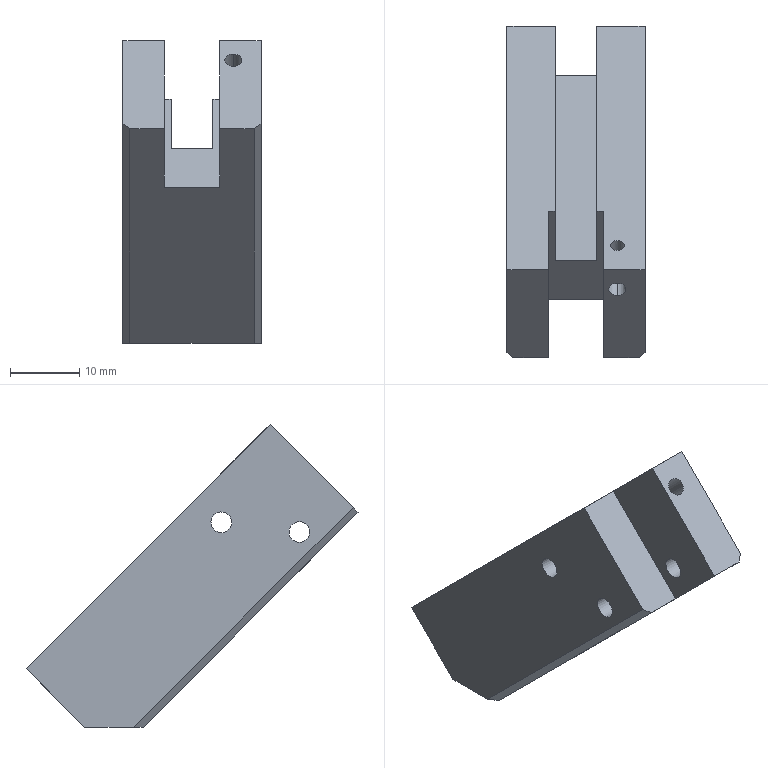Component | SolidWorks | ZL-10-07Slider-1 | 1 solid | 34 faces | box 20 x 48.08 x 43.84 mm | volume 13354 mm3 | plane 18 | cylinder 14 | cone 2 | commonest cylinder face diameters 3 x8 2 x4 2.5 x2
build123d program:
from build123d import *

# Parameters (mm, degrees)
EXTRUDE1_DEPTH        = 50
M3_TAPPED_HOLE1_D     = 2.5
M3_TAPPED_HOLE1_DEPTH = 7.5
M3_TAPPED_HOLE1_TIP   = 0.7511
SKETCH6_R             = 1
CUT_EXTRUDE1_DEPTH    = 6
CHAMFER1_SIZE         = 6
SKETCH7_R             = 1.5
CUT_EXTRUDE2_DEPTH    = 57.78
SKETCH8_W             = 8
SKETCH8_H             = 12
CUT_EXTRUDE3_DEPTH    = 55.074
SKETCH9_R             = 1.5
CUT_EXTRUDE4_DEPTH    = 57.78
CHAMFER2_SIZE         = 1


with BuildPart() as part:
    # Sketch1 → Extrude1 (new body)
    with BuildSketch(Plane(origin=(0, 0, 0), x_dir=(1, 0, 0), z_dir=(0, 1, 0))):
        Polygon((10, 0), (-10, 0), (-10, 18), (-3, 18), (-3, 8), (3, 8), (3, 18), (10, 18), align=None)
    extrude(amount=EXTRUDE1_DEPTH)

    # M3 Tapped Hole1
    with Locations(Plane.XZ):
        with Locations((-6, -14)):
            Hole(M3_TAPPED_HOLE1_D / 2, depth=M3_TAPPED_HOLE1_DEPTH)
            with Locations((0, 0, -(M3_TAPPED_HOLE1_DEPTH + M3_TAPPED_HOLE1_TIP / 2))):  # 118° drill point
                Cone(0, M3_TAPPED_HOLE1_D / 2, M3_TAPPED_HOLE1_TIP, mode=Mode.SUBTRACT)

    # Sketch6 → Cut-Extrude1 (cut)
    with BuildSketch(Plane(origin=(0, 0, -18), x_dir=(-1, 0, 0), z_dir=(0, 0, -1))):
        with Locations((6, 5)):
            Circle(SKETCH6_R)
    extrude(amount=-CUT_EXTRUDE1_DEPTH, mode=Mode.SUBTRACT)

    # Chamfer1
    chamfer1_edges = [part.edges().sort_by_distance(p)[0] for p in [
        (0, 50, 0),
    ]]
    chamfer(chamfer1_edges, length=CHAMFER1_SIZE)

    # Sketch7 → Cut-Extrude2 (cut, through all)
    with BuildSketch(Plane.ZY.offset(10)):
        with Locations((-13, 15)):
            Circle(SKETCH7_R)
    extrude(amount=-CUT_EXTRUDE2_DEPTH, mode=Mode.SUBTRACT)

    # Sketch8 → Cut-Extrude3 (cut, through all)
    with BuildSketch(Plane(origin=(0, 0, -18), x_dir=(-1, 0, 0), z_dir=(0, 0, -1))):
        with Locations((0, 6)):
            Rectangle(SKETCH8_W, SKETCH8_H)
    extrude(amount=-CUT_EXTRUDE3_DEPTH, mode=Mode.SUBTRACT)

    # Sketch9 → Cut-Extrude4 (cut, through all)
    with BuildSketch(Plane(origin=(10, 0, 0), x_dir=(0, 0, -1), z_dir=(1, 0, 0))):
        with Locations((4, 8)):
            Circle(SKETCH9_R)
    extrude(amount=-CUT_EXTRUDE4_DEPTH, mode=Mode.SUBTRACT)

    # Chamfer2
    chamfer2_edges = [part.edges().sort_by_distance(p)[0] for p in [
        (10, 22, 0),
        (-10, 22, 0),
    ]]
    chamfer(chamfer2_edges, length=CHAMFER2_SIZE)


solid = part.part

# Placed as in the assembly
solid = solid.moved(Location((42.823, 56.084, -16.405), (135, 0, -180)))